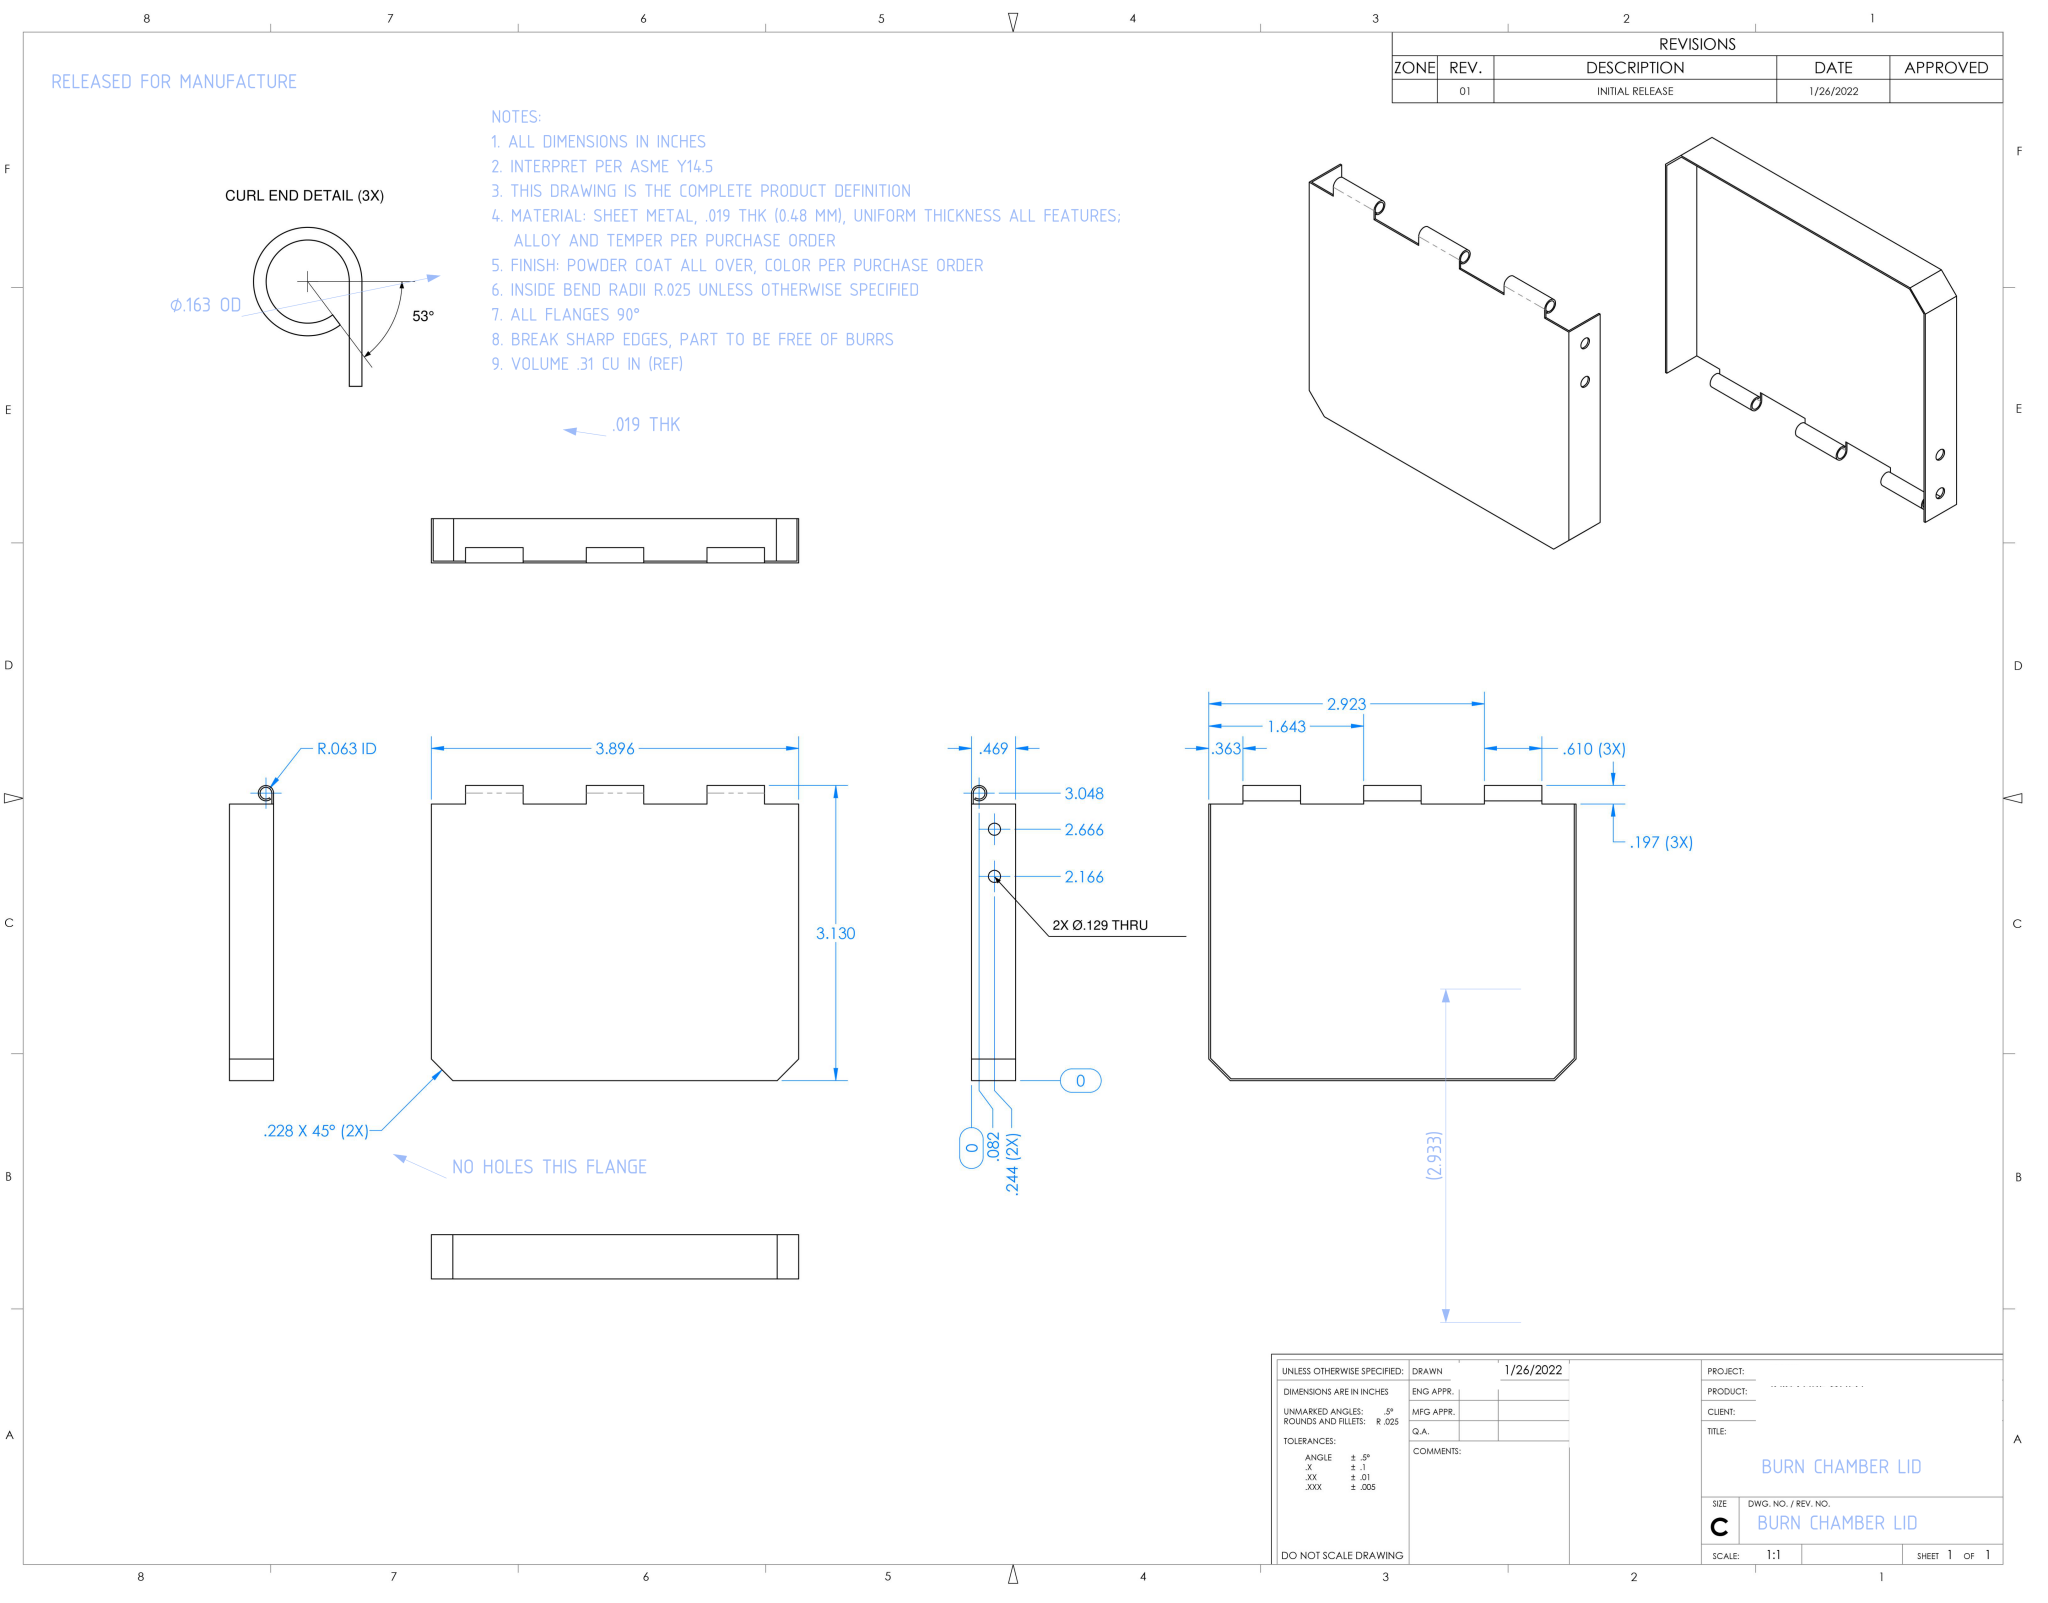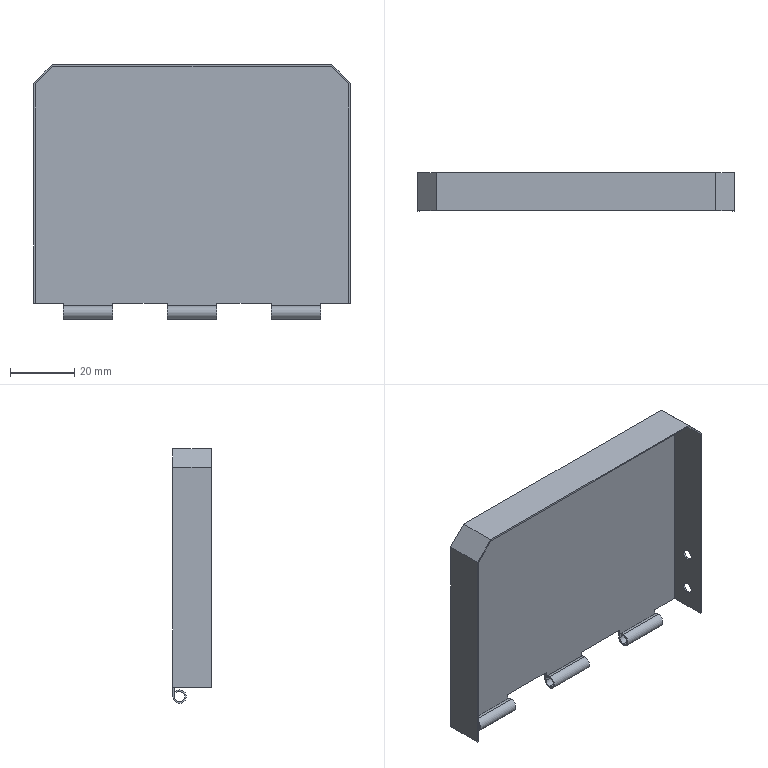Part | NX | drawing in metres | 1 solid | 48 faces | box 98.96 x 11.91 x 79.49 mm | volume 5145 mm3 | plane 26 | cylinder 22 | commonest cylinder face diameters 4.14 x9 3.175 x9 3.277 x4